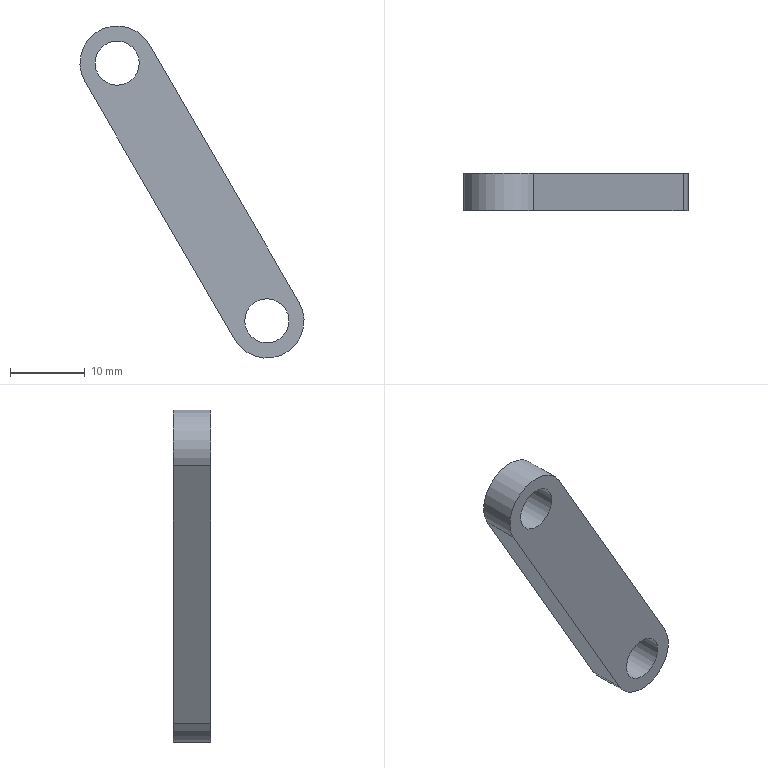Component | NX | 40 | 1 solid | 8 faces | box 30.09 x 5 x 44.59 mm | volume 2117 mm3 | plane 4 | cylinder 4 | commonest cylinder face diameters 10 x2 5.929 x2
STEP:
#1=CARTESIAN_POINT('',(0.,0.,0.));
#2=DIRECTION('',(0.,0.,1.));
#3=DIRECTION('',(1.,0.,0.));
#4=AXIS2_PLACEMENT_3D('',#1,#2,#3);
#5=CARTESIAN_POINT('',(-75.911,45.95,-2.511));
#6=VERTEX_POINT('',#5);
#7=CARTESIAN_POINT('',(-95.999,45.95,32.08));
#8=VERTEX_POINT('',#7);
#9=CARTESIAN_POINT('',(-75.911,45.95,-2.511));
#10=DIRECTION('',(-0.5022,0.,0.8648));
#11=VECTOR('',#10,1.);
#12=LINE('',#9,#11);
#13=CARTESIAN_POINT('',(-75.911,40.95,-2.511));
#14=DIRECTION('',(-0.8648,0.,-0.5022));
#15=DIRECTION('',(-0.5022,0.,0.8648));
#16=AXIS2_PLACEMENT_3D('',#13,#14,#15);
#17=PLANE('',#16);
#18=CARTESIAN_POINT('',(0.,5.));
#19=DIRECTION('',(1.,0.));
#20=VECTOR('',#19,1.);
#21=LINE('',#18,#20);
#22=(GEOMETRIC_REPRESENTATION_CONTEXT(2)PARAMETRIC_REPRESENTATION_CONTEXT()REPRESENTATION_CONTEXT('',''));
#23=DEFINITIONAL_REPRESENTATION('',(#21),#22);
#24=PCURVE('',#17,#23);
#25=CARTESIAN_POINT('',(-91.675,45.95,34.591));
#26=DIRECTION('',(0.,1.,0.));
#27=DIRECTION('',(-0.8648,0.,-0.5022));
#28=AXIS2_PLACEMENT_3D('',#25,#26,#27);
#29=PLANE('',#28);
#30=CARTESIAN_POINT('',(5.,-40.));
#31=DIRECTION('',(-0.,1.));
#32=VECTOR('',#31,1.);
#33=LINE('',#30,#32);
#34=(GEOMETRIC_REPRESENTATION_CONTEXT(2)PARAMETRIC_REPRESENTATION_CONTEXT()REPRESENTATION_CONTEXT('',''));
#35=DEFINITIONAL_REPRESENTATION('',(#33),#34);
#36=PCURVE('',#29,#35);
#37=SURFACE_CURVE('',#12,(#24,#36),.PCURVE_S1.);
#38=EDGE_CURVE('',#6,#8,#37,.T.);
#39=ORIENTED_EDGE('',*,*,#38,.F.);
#40=CARTESIAN_POINT('',(-75.911,40.95,-2.511));
#41=VERTEX_POINT('',#40);
#42=CARTESIAN_POINT('',(-75.911,40.95,-2.511));
#43=DIRECTION('',(0.,1.,0.));
#44=VECTOR('',#43,1.);
#45=LINE('',#42,#44);
#46=CARTESIAN_POINT('',(0.,0.));
#47=DIRECTION('',(0.,1.));
#48=VECTOR('',#47,1.);
#49=LINE('',#46,#48);
#50=(GEOMETRIC_REPRESENTATION_CONTEXT(2)PARAMETRIC_REPRESENTATION_CONTEXT()REPRESENTATION_CONTEXT('',''));
#51=DEFINITIONAL_REPRESENTATION('',(#49),#50);
#52=PCURVE('',#17,#51);
#53=CARTESIAN_POINT('',(-71.588,40.95,0.));
#54=DIRECTION('',(0.,1.,0.));
#55=DIRECTION('',(-0.8648,0.,-0.5022));
#56=AXIS2_PLACEMENT_3D('',#53,#54,#55);
#57=CYLINDRICAL_SURFACE('',#56,5.);
#58=CARTESIAN_POINT('',(6.283,0.));
#59=DIRECTION('',(0.,1.));
#60=VECTOR('',#59,1.);
#61=LINE('',#58,#60);
#62=(GEOMETRIC_REPRESENTATION_CONTEXT(2)PARAMETRIC_REPRESENTATION_CONTEXT()REPRESENTATION_CONTEXT('',''));
#63=DEFINITIONAL_REPRESENTATION('',(#61),#62);
#64=PCURVE('',#57,#63);
#65=SURFACE_CURVE('',#45,(#52,#64),.PCURVE_S1.);
#66=EDGE_CURVE('',#41,#6,#65,.T.);
#67=ORIENTED_EDGE('',*,*,#66,.F.);
#68=CARTESIAN_POINT('',(-95.999,40.95,32.08));
#69=VERTEX_POINT('',#68);
#70=CARTESIAN_POINT('',(-75.911,40.95,-2.511));
#71=DIRECTION('',(-0.5022,0.,0.8648));
#72=VECTOR('',#71,1.);
#73=LINE('',#70,#72);
#74=CARTESIAN_POINT('',(0.,0.));
#75=DIRECTION('',(1.,0.));
#76=VECTOR('',#75,1.);
#77=LINE('',#74,#76);
#78=(GEOMETRIC_REPRESENTATION_CONTEXT(2)PARAMETRIC_REPRESENTATION_CONTEXT()REPRESENTATION_CONTEXT('',''));
#79=DEFINITIONAL_REPRESENTATION('',(#77),#78);
#80=PCURVE('',#17,#79);
#81=CARTESIAN_POINT('',(-91.675,40.95,34.591));
#82=DIRECTION('',(0.,1.,0.));
#83=DIRECTION('',(-0.8648,0.,-0.5022));
#84=AXIS2_PLACEMENT_3D('',#81,#82,#83);
#85=PLANE('',#84);
#86=CARTESIAN_POINT('',(5.,-40.));
#87=DIRECTION('',(-0.,1.));
#88=VECTOR('',#87,1.);
#89=LINE('',#86,#88);
#90=(GEOMETRIC_REPRESENTATION_CONTEXT(2)PARAMETRIC_REPRESENTATION_CONTEXT()REPRESENTATION_CONTEXT('',''));
#91=DEFINITIONAL_REPRESENTATION('',(#89),#90);
#92=PCURVE('',#85,#91);
#93=SURFACE_CURVE('',#73,(#80,#92),.PCURVE_S1.);
#94=EDGE_CURVE('',#41,#69,#93,.T.);
#95=ORIENTED_EDGE('',*,*,#94,.T.);
#96=CARTESIAN_POINT('',(-95.999,40.95,32.08));
#97=DIRECTION('',(0.,1.,0.));
#98=VECTOR('',#97,1.);
#99=LINE('',#96,#98);
#100=CARTESIAN_POINT('',(40.,0.));
#101=DIRECTION('',(0.,1.));
#102=VECTOR('',#101,1.);
#103=LINE('',#100,#102);
#104=(GEOMETRIC_REPRESENTATION_CONTEXT(2)PARAMETRIC_REPRESENTATION_CONTEXT()REPRESENTATION_CONTEXT('',''));
#105=DEFINITIONAL_REPRESENTATION('',(#103),#104);
#106=PCURVE('',#17,#105);
#107=CARTESIAN_POINT('',(-91.675,40.95,34.591));
#108=DIRECTION('',(0.,1.,0.));
#109=DIRECTION('',(-0.8648,0.,-0.5022));
#110=AXIS2_PLACEMENT_3D('',#107,#108,#109);
#111=CYLINDRICAL_SURFACE('',#110,5.);
#112=CARTESIAN_POINT('',(0.,0.));
#113=DIRECTION('',(0.,1.));
#114=VECTOR('',#113,1.);
#115=LINE('',#112,#114);
#116=(GEOMETRIC_REPRESENTATION_CONTEXT(2)PARAMETRIC_REPRESENTATION_CONTEXT()REPRESENTATION_CONTEXT('',''));
#117=DEFINITIONAL_REPRESENTATION('',(#115),#116);
#118=PCURVE('',#111,#117);
#119=SURFACE_CURVE('',#99,(#106,#118),.PCURVE_S1.);
#120=EDGE_CURVE('',#69,#8,#119,.T.);
#121=ORIENTED_EDGE('',*,*,#120,.T.);
#122=EDGE_LOOP('',(#39,#67,#95,#121));
#123=FACE_BOUND('',#122,.T.);
#124=ADVANCED_FACE('',(#123),#17,.T.);
#125=CARTESIAN_POINT('',(-87.351,45.95,37.101));
#126=VERTEX_POINT('',#125);
#127=CARTESIAN_POINT('',(-91.675,45.95,34.591));
#128=DIRECTION('',(0.,1.,0.));
#129=DIRECTION('',(-0.8648,0.,-0.5022));
#130=AXIS2_PLACEMENT_3D('',#127,#128,#129);
#131=CIRCLE('',#130,5.);
#132=CARTESIAN_POINT('',(0.,5.));
#133=DIRECTION('',(1.,0.));
#134=VECTOR('',#133,1.);
#135=LINE('',#132,#134);
#136=(GEOMETRIC_REPRESENTATION_CONTEXT(2)PARAMETRIC_REPRESENTATION_CONTEXT()REPRESENTATION_CONTEXT('',''));
#137=DEFINITIONAL_REPRESENTATION('',(#135),#136);
#138=PCURVE('',#111,#137);
#139=CARTESIAN_POINT('',(0.,0.));
#140=DIRECTION('',(1.,0.));
#141=AXIS2_PLACEMENT_2D('',#139,#140);
#142=CIRCLE('',#141,5.);
#143=(GEOMETRIC_REPRESENTATION_CONTEXT(2)PARAMETRIC_REPRESENTATION_CONTEXT()REPRESENTATION_CONTEXT('',''));
#144=DEFINITIONAL_REPRESENTATION('',(#142),#143);
#145=PCURVE('',#29,#144);
#146=SURFACE_CURVE('',#131,(#138,#145),.PCURVE_S1.);
#147=EDGE_CURVE('',#8,#126,#146,.T.);
#148=ORIENTED_EDGE('',*,*,#147,.F.);
#149=ORIENTED_EDGE('',*,*,#120,.F.);
#150=CARTESIAN_POINT('',(-87.351,40.95,37.101));
#151=VERTEX_POINT('',#150);
#152=CARTESIAN_POINT('',(-91.675,40.95,34.591));
#153=DIRECTION('',(0.,1.,0.));
#154=DIRECTION('',(-0.8648,0.,-0.5022));
#155=AXIS2_PLACEMENT_3D('',#152,#153,#154);
#156=CIRCLE('',#155,5.);
#157=CARTESIAN_POINT('',(0.,0.));
#158=DIRECTION('',(1.,0.));
#159=VECTOR('',#158,1.);
#160=LINE('',#157,#159);
#161=(GEOMETRIC_REPRESENTATION_CONTEXT(2)PARAMETRIC_REPRESENTATION_CONTEXT()REPRESENTATION_CONTEXT('',''));
#162=DEFINITIONAL_REPRESENTATION('',(#160),#161);
#163=PCURVE('',#111,#162);
#164=CARTESIAN_POINT('',(0.,0.));
#165=DIRECTION('',(1.,0.));
#166=AXIS2_PLACEMENT_2D('',#164,#165);
#167=CIRCLE('',#166,5.);
#168=(GEOMETRIC_REPRESENTATION_CONTEXT(2)PARAMETRIC_REPRESENTATION_CONTEXT()REPRESENTATION_CONTEXT('',''));
#169=DEFINITIONAL_REPRESENTATION('',(#167),#168);
#170=PCURVE('',#85,#169);
#171=SURFACE_CURVE('',#156,(#163,#170),.PCURVE_S1.);
#172=EDGE_CURVE('',#69,#151,#171,.T.);
#173=ORIENTED_EDGE('',*,*,#172,.T.);
#174=CARTESIAN_POINT('',(-87.351,40.95,37.101));
#175=DIRECTION('',(0.,1.,0.));
#176=VECTOR('',#175,1.);
#177=LINE('',#174,#176);
#178=CARTESIAN_POINT('',(3.142,0.));
#179=DIRECTION('',(0.,1.));
#180=VECTOR('',#179,1.);
#181=LINE('',#178,#180);
#182=(GEOMETRIC_REPRESENTATION_CONTEXT(2)PARAMETRIC_REPRESENTATION_CONTEXT()REPRESENTATION_CONTEXT('',''));
#183=DEFINITIONAL_REPRESENTATION('',(#181),#182);
#184=PCURVE('',#111,#183);
#185=CARTESIAN_POINT('',(-87.351,40.95,37.101));
#186=DIRECTION('',(0.8648,0.,0.5022));
#187=DIRECTION('',(0.5022,0.,-0.8648));
#188=AXIS2_PLACEMENT_3D('',#185,#186,#187);
#189=PLANE('',#188);
#190=CARTESIAN_POINT('',(0.,0.));
#191=DIRECTION('',(0.,1.));
#192=VECTOR('',#191,1.);
#193=LINE('',#190,#192);
#194=(GEOMETRIC_REPRESENTATION_CONTEXT(2)PARAMETRIC_REPRESENTATION_CONTEXT()REPRESENTATION_CONTEXT('',''));
#195=DEFINITIONAL_REPRESENTATION('',(#193),#194);
#196=PCURVE('',#189,#195);
#197=SURFACE_CURVE('',#177,(#184,#196),.PCURVE_S1.);
#198=EDGE_CURVE('',#151,#126,#197,.T.);
#199=ORIENTED_EDGE('',*,*,#198,.T.);
#200=EDGE_LOOP('',(#148,#149,#173,#199));
#201=FACE_BOUND('',#200,.T.);
#202=ADVANCED_FACE('',(#201),#111,.T.);
#203=CARTESIAN_POINT('',(-67.264,45.95,2.511));
#204=VERTEX_POINT('',#203);
#205=CARTESIAN_POINT('',(-87.351,45.95,37.101));
#206=DIRECTION('',(0.5022,0.,-0.8648));
#207=VECTOR('',#206,1.);
#208=LINE('',#205,#207);
#209=CARTESIAN_POINT('',(0.,5.));
#210=DIRECTION('',(1.,0.));
#211=VECTOR('',#210,1.);
#212=LINE('',#209,#211);
#213=(GEOMETRIC_REPRESENTATION_CONTEXT(2)PARAMETRIC_REPRESENTATION_CONTEXT()REPRESENTATION_CONTEXT('',''));
#214=DEFINITIONAL_REPRESENTATION('',(#212),#213);
#215=PCURVE('',#189,#214);
#216=CARTESIAN_POINT('',(-5.,0.));
#217=DIRECTION('',(0.,-1.));
#218=VECTOR('',#217,1.);
#219=LINE('',#216,#218);
#220=(GEOMETRIC_REPRESENTATION_CONTEXT(2)PARAMETRIC_REPRESENTATION_CONTEXT()REPRESENTATION_CONTEXT('',''));
#221=DEFINITIONAL_REPRESENTATION('',(#219),#220);
#222=PCURVE('',#29,#221);
#223=SURFACE_CURVE('',#208,(#215,#222),.PCURVE_S1.);
#224=EDGE_CURVE('',#126,#204,#223,.T.);
#225=ORIENTED_EDGE('',*,*,#224,.F.);
#226=ORIENTED_EDGE('',*,*,#198,.F.);
#227=CARTESIAN_POINT('',(-67.264,40.95,2.511));
#228=VERTEX_POINT('',#227);
#229=CARTESIAN_POINT('',(-87.351,40.95,37.101));
#230=DIRECTION('',(0.5022,0.,-0.8648));
#231=VECTOR('',#230,1.);
#232=LINE('',#229,#231);
#233=CARTESIAN_POINT('',(0.,0.));
#234=DIRECTION('',(1.,0.));
#235=VECTOR('',#234,1.);
#236=LINE('',#233,#235);
#237=(GEOMETRIC_REPRESENTATION_CONTEXT(2)PARAMETRIC_REPRESENTATION_CONTEXT()REPRESENTATION_CONTEXT('',''));
#238=DEFINITIONAL_REPRESENTATION('',(#236),#237);
#239=PCURVE('',#189,#238);
#240=CARTESIAN_POINT('',(-5.,0.));
#241=DIRECTION('',(0.,-1.));
#242=VECTOR('',#241,1.);
#243=LINE('',#240,#242);
#244=(GEOMETRIC_REPRESENTATION_CONTEXT(2)PARAMETRIC_REPRESENTATION_CONTEXT()REPRESENTATION_CONTEXT('',''));
#245=DEFINITIONAL_REPRESENTATION('',(#243),#244);
#246=PCURVE('',#85,#245);
#247=SURFACE_CURVE('',#232,(#239,#246),.PCURVE_S1.);
#248=EDGE_CURVE('',#151,#228,#247,.T.);
#249=ORIENTED_EDGE('',*,*,#248,.T.);
#250=CARTESIAN_POINT('',(-67.264,40.95,2.511));
#251=DIRECTION('',(0.,1.,0.));
#252=VECTOR('',#251,1.);
#253=LINE('',#250,#252);
#254=CARTESIAN_POINT('',(40.,0.));
#255=DIRECTION('',(0.,1.));
#256=VECTOR('',#255,1.);
#257=LINE('',#254,#256);
#258=(GEOMETRIC_REPRESENTATION_CONTEXT(2)PARAMETRIC_REPRESENTATION_CONTEXT()REPRESENTATION_CONTEXT('',''));
#259=DEFINITIONAL_REPRESENTATION('',(#257),#258);
#260=PCURVE('',#189,#259);
#261=CARTESIAN_POINT('',(3.142,0.));
#262=DIRECTION('',(0.,1.));
#263=VECTOR('',#262,1.);
#264=LINE('',#261,#263);
#265=(GEOMETRIC_REPRESENTATION_CONTEXT(2)PARAMETRIC_REPRESENTATION_CONTEXT()REPRESENTATION_CONTEXT('',''));
#266=DEFINITIONAL_REPRESENTATION('',(#264),#265);
#267=PCURVE('',#57,#266);
#268=SURFACE_CURVE('',#253,(#260,#267),.PCURVE_S1.);
#269=EDGE_CURVE('',#228,#204,#268,.T.);
#270=ORIENTED_EDGE('',*,*,#269,.T.);
#271=EDGE_LOOP('',(#225,#226,#249,#270));
#272=FACE_BOUND('',#271,.T.);
#273=ADVANCED_FACE('',(#272),#189,.T.);
#274=CARTESIAN_POINT('',(-74.151,40.95,-1.489));
#275=VERTEX_POINT('',#274);
#276=CARTESIAN_POINT('',(-71.588,40.95,0.));
#277=DIRECTION('',(0.,1.,0.));
#278=DIRECTION('',(-0.8648,0.,-0.5022));
#279=AXIS2_PLACEMENT_3D('',#276,#277,#278);
#280=CIRCLE('',#279,2.964);
#281=CARTESIAN_POINT('',(-71.588,40.95,0.));
#282=DIRECTION('',(0.,1.,0.));
#283=DIRECTION('',(-0.8648,0.,-0.5022));
#284=AXIS2_PLACEMENT_3D('',#281,#282,#283);
#285=CYLINDRICAL_SURFACE('',#284,2.964);
#286=CARTESIAN_POINT('',(0.,0.));
#287=DIRECTION('',(1.,0.));
#288=VECTOR('',#287,1.);
#289=LINE('',#286,#288);
#290=(GEOMETRIC_REPRESENTATION_CONTEXT(2)PARAMETRIC_REPRESENTATION_CONTEXT()REPRESENTATION_CONTEXT('',''));
#291=DEFINITIONAL_REPRESENTATION('',(#289),#290);
#292=PCURVE('',#285,#291);
#293=CARTESIAN_POINT('',(-0.,-40.));
#294=DIRECTION('',(1.,-0.));
#295=AXIS2_PLACEMENT_2D('',#293,#294);
#296=CIRCLE('',#295,2.964);
#297=(GEOMETRIC_REPRESENTATION_CONTEXT(2)PARAMETRIC_REPRESENTATION_CONTEXT()REPRESENTATION_CONTEXT('',''));
#298=DEFINITIONAL_REPRESENTATION('',(#296),#297);
#299=PCURVE('',#85,#298);
#300=SURFACE_CURVE('',#280,(#292,#299),.PCURVE_S1.);
#301=EDGE_CURVE('',#275,#275,#300,.T.);
#302=ORIENTED_EDGE('',*,*,#301,.T.);
#303=CARTESIAN_POINT('',(-74.151,45.95,-1.489));
#304=VERTEX_POINT('',#303);
#305=CARTESIAN_POINT('',(-74.151,40.95,-1.489));
#306=CARTESIAN_POINT('',(-74.151,45.95,-1.489));
#307=B_SPLINE_CURVE_WITH_KNOTS('',1,(#305,#306),.UNSPECIFIED.,.F.,.F.,(2,2),(0.,5.),.PIECEWISE_BEZIER_KNOTS.);
#308=CARTESIAN_POINT('',(6.283,0.));
#309=DIRECTION('',(0.,1.));
#310=VECTOR('',#309,1.);
#311=LINE('',#308,#310);
#312=(GEOMETRIC_REPRESENTATION_CONTEXT(2)PARAMETRIC_REPRESENTATION_CONTEXT()REPRESENTATION_CONTEXT('',''));
#313=DEFINITIONAL_REPRESENTATION('',(#311),#312);
#314=PCURVE('',#285,#313);
#315=CARTESIAN_POINT('',(0.,0.));
#316=DIRECTION('',(0.,1.));
#317=VECTOR('',#316,1.);
#318=LINE('',#315,#317);
#319=(GEOMETRIC_REPRESENTATION_CONTEXT(2)PARAMETRIC_REPRESENTATION_CONTEXT()REPRESENTATION_CONTEXT('',''));
#320=DEFINITIONAL_REPRESENTATION('',(#318),#319);
#321=PCURVE('',#285,#320);
#322=SEAM_CURVE('',#307,(#314,#321),.PCURVE_S1.);
#323=EDGE_CURVE('',#275,#304,#322,.T.);
#324=ORIENTED_EDGE('',*,*,#323,.T.);
#325=CARTESIAN_POINT('',(-71.588,45.95,0.));
#326=DIRECTION('',(0.,1.,0.));
#327=DIRECTION('',(-0.8648,0.,-0.5022));
#328=AXIS2_PLACEMENT_3D('',#325,#326,#327);
#329=CIRCLE('',#328,2.964);
#330=CARTESIAN_POINT('',(0.,5.));
#331=DIRECTION('',(1.,0.));
#332=VECTOR('',#331,1.);
#333=LINE('',#330,#332);
#334=(GEOMETRIC_REPRESENTATION_CONTEXT(2)PARAMETRIC_REPRESENTATION_CONTEXT()REPRESENTATION_CONTEXT('',''));
#335=DEFINITIONAL_REPRESENTATION('',(#333),#334);
#336=PCURVE('',#285,#335);
#337=CARTESIAN_POINT('',(-0.,-40.));
#338=DIRECTION('',(1.,-0.));
#339=AXIS2_PLACEMENT_2D('',#337,#338);
#340=CIRCLE('',#339,2.964);
#341=(GEOMETRIC_REPRESENTATION_CONTEXT(2)PARAMETRIC_REPRESENTATION_CONTEXT()REPRESENTATION_CONTEXT('',''));
#342=DEFINITIONAL_REPRESENTATION('',(#340),#341);
#343=PCURVE('',#29,#342);
#344=SURFACE_CURVE('',#329,(#336,#343),.PCURVE_S1.);
#345=EDGE_CURVE('',#304,#304,#344,.T.);
#346=ORIENTED_EDGE('',*,*,#345,.F.);
#347=ORIENTED_EDGE('',*,*,#323,.F.);
#348=EDGE_LOOP('',(#302,#324,#346,#347));
#349=FACE_BOUND('',#348,.F.);
#350=ADVANCED_FACE('',(#349),#285,.F.);
#351=CARTESIAN_POINT('',(-71.588,45.95,0.));
#352=DIRECTION('',(0.,1.,0.));
#353=DIRECTION('',(-0.8648,0.,-0.5022));
#354=AXIS2_PLACEMENT_3D('',#351,#352,#353);
#355=CIRCLE('',#354,5.);
#356=CARTESIAN_POINT('',(0.,5.));
#357=DIRECTION('',(1.,0.));
#358=VECTOR('',#357,1.);
#359=LINE('',#356,#358);
#360=(GEOMETRIC_REPRESENTATION_CONTEXT(2)PARAMETRIC_REPRESENTATION_CONTEXT()REPRESENTATION_CONTEXT('',''));
#361=DEFINITIONAL_REPRESENTATION('',(#359),#360);
#362=PCURVE('',#57,#361);
#363=CARTESIAN_POINT('',(-0.,-40.));
#364=DIRECTION('',(1.,0.));
#365=AXIS2_PLACEMENT_2D('',#363,#364);
#366=CIRCLE('',#365,5.);
#367=(GEOMETRIC_REPRESENTATION_CONTEXT(2)PARAMETRIC_REPRESENTATION_CONTEXT()REPRESENTATION_CONTEXT('',''));
#368=DEFINITIONAL_REPRESENTATION('',(#366),#367);
#369=PCURVE('',#29,#368);
#370=SURFACE_CURVE('',#355,(#362,#369),.PCURVE_S1.);
#371=EDGE_CURVE('',#204,#6,#370,.T.);
#372=ORIENTED_EDGE('',*,*,#371,.F.);
#373=ORIENTED_EDGE('',*,*,#269,.F.);
#374=CARTESIAN_POINT('',(-71.588,40.95,0.));
#375=DIRECTION('',(0.,1.,0.));
#376=DIRECTION('',(-0.8648,0.,-0.5022));
#377=AXIS2_PLACEMENT_3D('',#374,#375,#376);
#378=CIRCLE('',#377,5.);
#379=CARTESIAN_POINT('',(0.,0.));
#380=DIRECTION('',(1.,0.));
#381=VECTOR('',#380,1.);
#382=LINE('',#379,#381);
#383=(GEOMETRIC_REPRESENTATION_CONTEXT(2)PARAMETRIC_REPRESENTATION_CONTEXT()REPRESENTATION_CONTEXT('',''));
#384=DEFINITIONAL_REPRESENTATION('',(#382),#383);
#385=PCURVE('',#57,#384);
#386=CARTESIAN_POINT('',(-0.,-40.));
#387=DIRECTION('',(1.,0.));
#388=AXIS2_PLACEMENT_2D('',#386,#387);
#389=CIRCLE('',#388,5.);
#390=(GEOMETRIC_REPRESENTATION_CONTEXT(2)PARAMETRIC_REPRESENTATION_CONTEXT()REPRESENTATION_CONTEXT('',''));
#391=DEFINITIONAL_REPRESENTATION('',(#389),#390);
#392=PCURVE('',#85,#391);
#393=SURFACE_CURVE('',#378,(#385,#392),.PCURVE_S1.);
#394=EDGE_CURVE('',#228,#41,#393,.T.);
#395=ORIENTED_EDGE('',*,*,#394,.T.);
#396=ORIENTED_EDGE('',*,*,#66,.T.);
#397=EDGE_LOOP('',(#372,#373,#395,#396));
#398=FACE_BOUND('',#397,.T.);
#399=ADVANCED_FACE('',(#398),#57,.T.);
#400=CARTESIAN_POINT('',(-94.238,40.95,33.102));
#401=VERTEX_POINT('',#400);
#402=CARTESIAN_POINT('',(-91.675,40.95,34.591));
#403=DIRECTION('',(0.,1.,0.));
#404=DIRECTION('',(-0.8648,0.,-0.5022));
#405=AXIS2_PLACEMENT_3D('',#402,#403,#404);
#406=CIRCLE('',#405,2.964);
#407=CARTESIAN_POINT('',(-91.675,40.95,34.591));
#408=DIRECTION('',(0.,1.,0.));
#409=DIRECTION('',(-0.8648,0.,-0.5022));
#410=AXIS2_PLACEMENT_3D('',#407,#408,#409);
#411=CYLINDRICAL_SURFACE('',#410,2.964);
#412=CARTESIAN_POINT('',(0.,0.));
#413=DIRECTION('',(1.,0.));
#414=VECTOR('',#413,1.);
#415=LINE('',#412,#414);
#416=(GEOMETRIC_REPRESENTATION_CONTEXT(2)PARAMETRIC_REPRESENTATION_CONTEXT()REPRESENTATION_CONTEXT('',''));
#417=DEFINITIONAL_REPRESENTATION('',(#415),#416);
#418=PCURVE('',#411,#417);
#419=CARTESIAN_POINT('',(0.,0.));
#420=DIRECTION('',(1.,-0.));
#421=AXIS2_PLACEMENT_2D('',#419,#420);
#422=CIRCLE('',#421,2.964);
#423=(GEOMETRIC_REPRESENTATION_CONTEXT(2)PARAMETRIC_REPRESENTATION_CONTEXT()REPRESENTATION_CONTEXT('',''));
#424=DEFINITIONAL_REPRESENTATION('',(#422),#423);
#425=PCURVE('',#85,#424);
#426=SURFACE_CURVE('',#406,(#418,#425),.PCURVE_S1.);
#427=EDGE_CURVE('',#401,#401,#426,.T.);
#428=ORIENTED_EDGE('',*,*,#427,.T.);
#429=CARTESIAN_POINT('',(-94.238,45.95,33.102));
#430=VERTEX_POINT('',#429);
#431=CARTESIAN_POINT('',(-94.238,40.95,33.102));
#432=CARTESIAN_POINT('',(-94.238,45.95,33.102));
#433=B_SPLINE_CURVE_WITH_KNOTS('',1,(#431,#432),.UNSPECIFIED.,.F.,.F.,(2,2),(0.,5.),.PIECEWISE_BEZIER_KNOTS.);
#434=CARTESIAN_POINT('',(6.283,0.));
#435=DIRECTION('',(0.,1.));
#436=VECTOR('',#435,1.);
#437=LINE('',#434,#436);
#438=(GEOMETRIC_REPRESENTATION_CONTEXT(2)PARAMETRIC_REPRESENTATION_CONTEXT()REPRESENTATION_CONTEXT('',''));
#439=DEFINITIONAL_REPRESENTATION('',(#437),#438);
#440=PCURVE('',#411,#439);
#441=CARTESIAN_POINT('',(0.,0.));
#442=DIRECTION('',(0.,1.));
#443=VECTOR('',#442,1.);
#444=LINE('',#441,#443);
#445=(GEOMETRIC_REPRESENTATION_CONTEXT(2)PARAMETRIC_REPRESENTATION_CONTEXT()REPRESENTATION_CONTEXT('',''));
#446=DEFINITIONAL_REPRESENTATION('',(#444),#445);
#447=PCURVE('',#411,#446);
#448=SEAM_CURVE('',#433,(#440,#447),.PCURVE_S1.);
#449=EDGE_CURVE('',#401,#430,#448,.T.);
#450=ORIENTED_EDGE('',*,*,#449,.T.);
#451=CARTESIAN_POINT('',(-91.675,45.95,34.591));
#452=DIRECTION('',(0.,1.,0.));
#453=DIRECTION('',(-0.8648,0.,-0.5022));
#454=AXIS2_PLACEMENT_3D('',#451,#452,#453);
#455=CIRCLE('',#454,2.964);
#456=CARTESIAN_POINT('',(0.,5.));
#457=DIRECTION('',(1.,0.));
#458=VECTOR('',#457,1.);
#459=LINE('',#456,#458);
#460=(GEOMETRIC_REPRESENTATION_CONTEXT(2)PARAMETRIC_REPRESENTATION_CONTEXT()REPRESENTATION_CONTEXT('',''));
#461=DEFINITIONAL_REPRESENTATION('',(#459),#460);
#462=PCURVE('',#411,#461);
#463=CARTESIAN_POINT('',(0.,0.));
#464=DIRECTION('',(1.,-0.));
#465=AXIS2_PLACEMENT_2D('',#463,#464);
#466=CIRCLE('',#465,2.964);
#467=(GEOMETRIC_REPRESENTATION_CONTEXT(2)PARAMETRIC_REPRESENTATION_CONTEXT()REPRESENTATION_CONTEXT('',''));
#468=DEFINITIONAL_REPRESENTATION('',(#466),#467);
#469=PCURVE('',#29,#468);
#470=SURFACE_CURVE('',#455,(#462,#469),.PCURVE_S1.);
#471=EDGE_CURVE('',#430,#430,#470,.T.);
#472=ORIENTED_EDGE('',*,*,#471,.F.);
#473=ORIENTED_EDGE('',*,*,#449,.F.);
#474=EDGE_LOOP('',(#428,#450,#472,#473));
#475=FACE_BOUND('',#474,.F.);
#476=ADVANCED_FACE('',(#475),#411,.F.);
#477=ORIENTED_EDGE('',*,*,#94,.F.);
#478=ORIENTED_EDGE('',*,*,#394,.F.);
#479=ORIENTED_EDGE('',*,*,#248,.F.);
#480=ORIENTED_EDGE('',*,*,#172,.F.);
#481=EDGE_LOOP('',(#477,#478,#479,#480));
#482=FACE_BOUND('',#481,.T.);
#483=ORIENTED_EDGE('',*,*,#301,.T.);
#484=EDGE_LOOP('',(#483));
#485=FACE_BOUND('',#484,.T.);
#486=ORIENTED_EDGE('',*,*,#427,.T.);
#487=EDGE_LOOP('',(#486));
#488=FACE_BOUND('',#487,.T.);
#489=ADVANCED_FACE('',(#482,#485,#488),#85,.F.);
#490=ORIENTED_EDGE('',*,*,#38,.T.);
#491=ORIENTED_EDGE('',*,*,#147,.T.);
#492=ORIENTED_EDGE('',*,*,#224,.T.);
#493=ORIENTED_EDGE('',*,*,#371,.T.);
#494=EDGE_LOOP('',(#490,#491,#492,#493));
#495=FACE_BOUND('',#494,.T.);
#496=ORIENTED_EDGE('',*,*,#345,.F.);
#497=EDGE_LOOP('',(#496));
#498=FACE_BOUND('',#497,.T.);
#499=ORIENTED_EDGE('',*,*,#471,.F.);
#500=EDGE_LOOP('',(#499));
#501=FACE_BOUND('',#500,.T.);
#502=ADVANCED_FACE('',(#495,#498,#501),#29,.T.);
#503=CLOSED_SHELL('',(#124,#202,#273,#350,#399,#476,#489,#502));
#504=MANIFOLD_SOLID_BREP('',#503);
#505=(LENGTH_UNIT()NAMED_UNIT(*)SI_UNIT(.MILLI.,.METRE.));
#506=UNCERTAINTY_MEASURE_WITH_UNIT(LENGTH_MEASURE(0.000002),#505,'','');
#507=(NAMED_UNIT(*)PLANE_ANGLE_UNIT()SI_UNIT($,.RADIAN.));
#508=(NAMED_UNIT(*)SI_UNIT($,.STERADIAN.)SOLID_ANGLE_UNIT());
#509=(GEOMETRIC_REPRESENTATION_CONTEXT(3)GLOBAL_UNCERTAINTY_ASSIGNED_CONTEXT((#506))GLOBAL_UNIT_ASSIGNED_CONTEXT((#505,#507,#508))REPRESENTATION_CONTEXT('',''));
#510=ADVANCED_BREP_SHAPE_REPRESENTATION('',(#4,#504),#509);